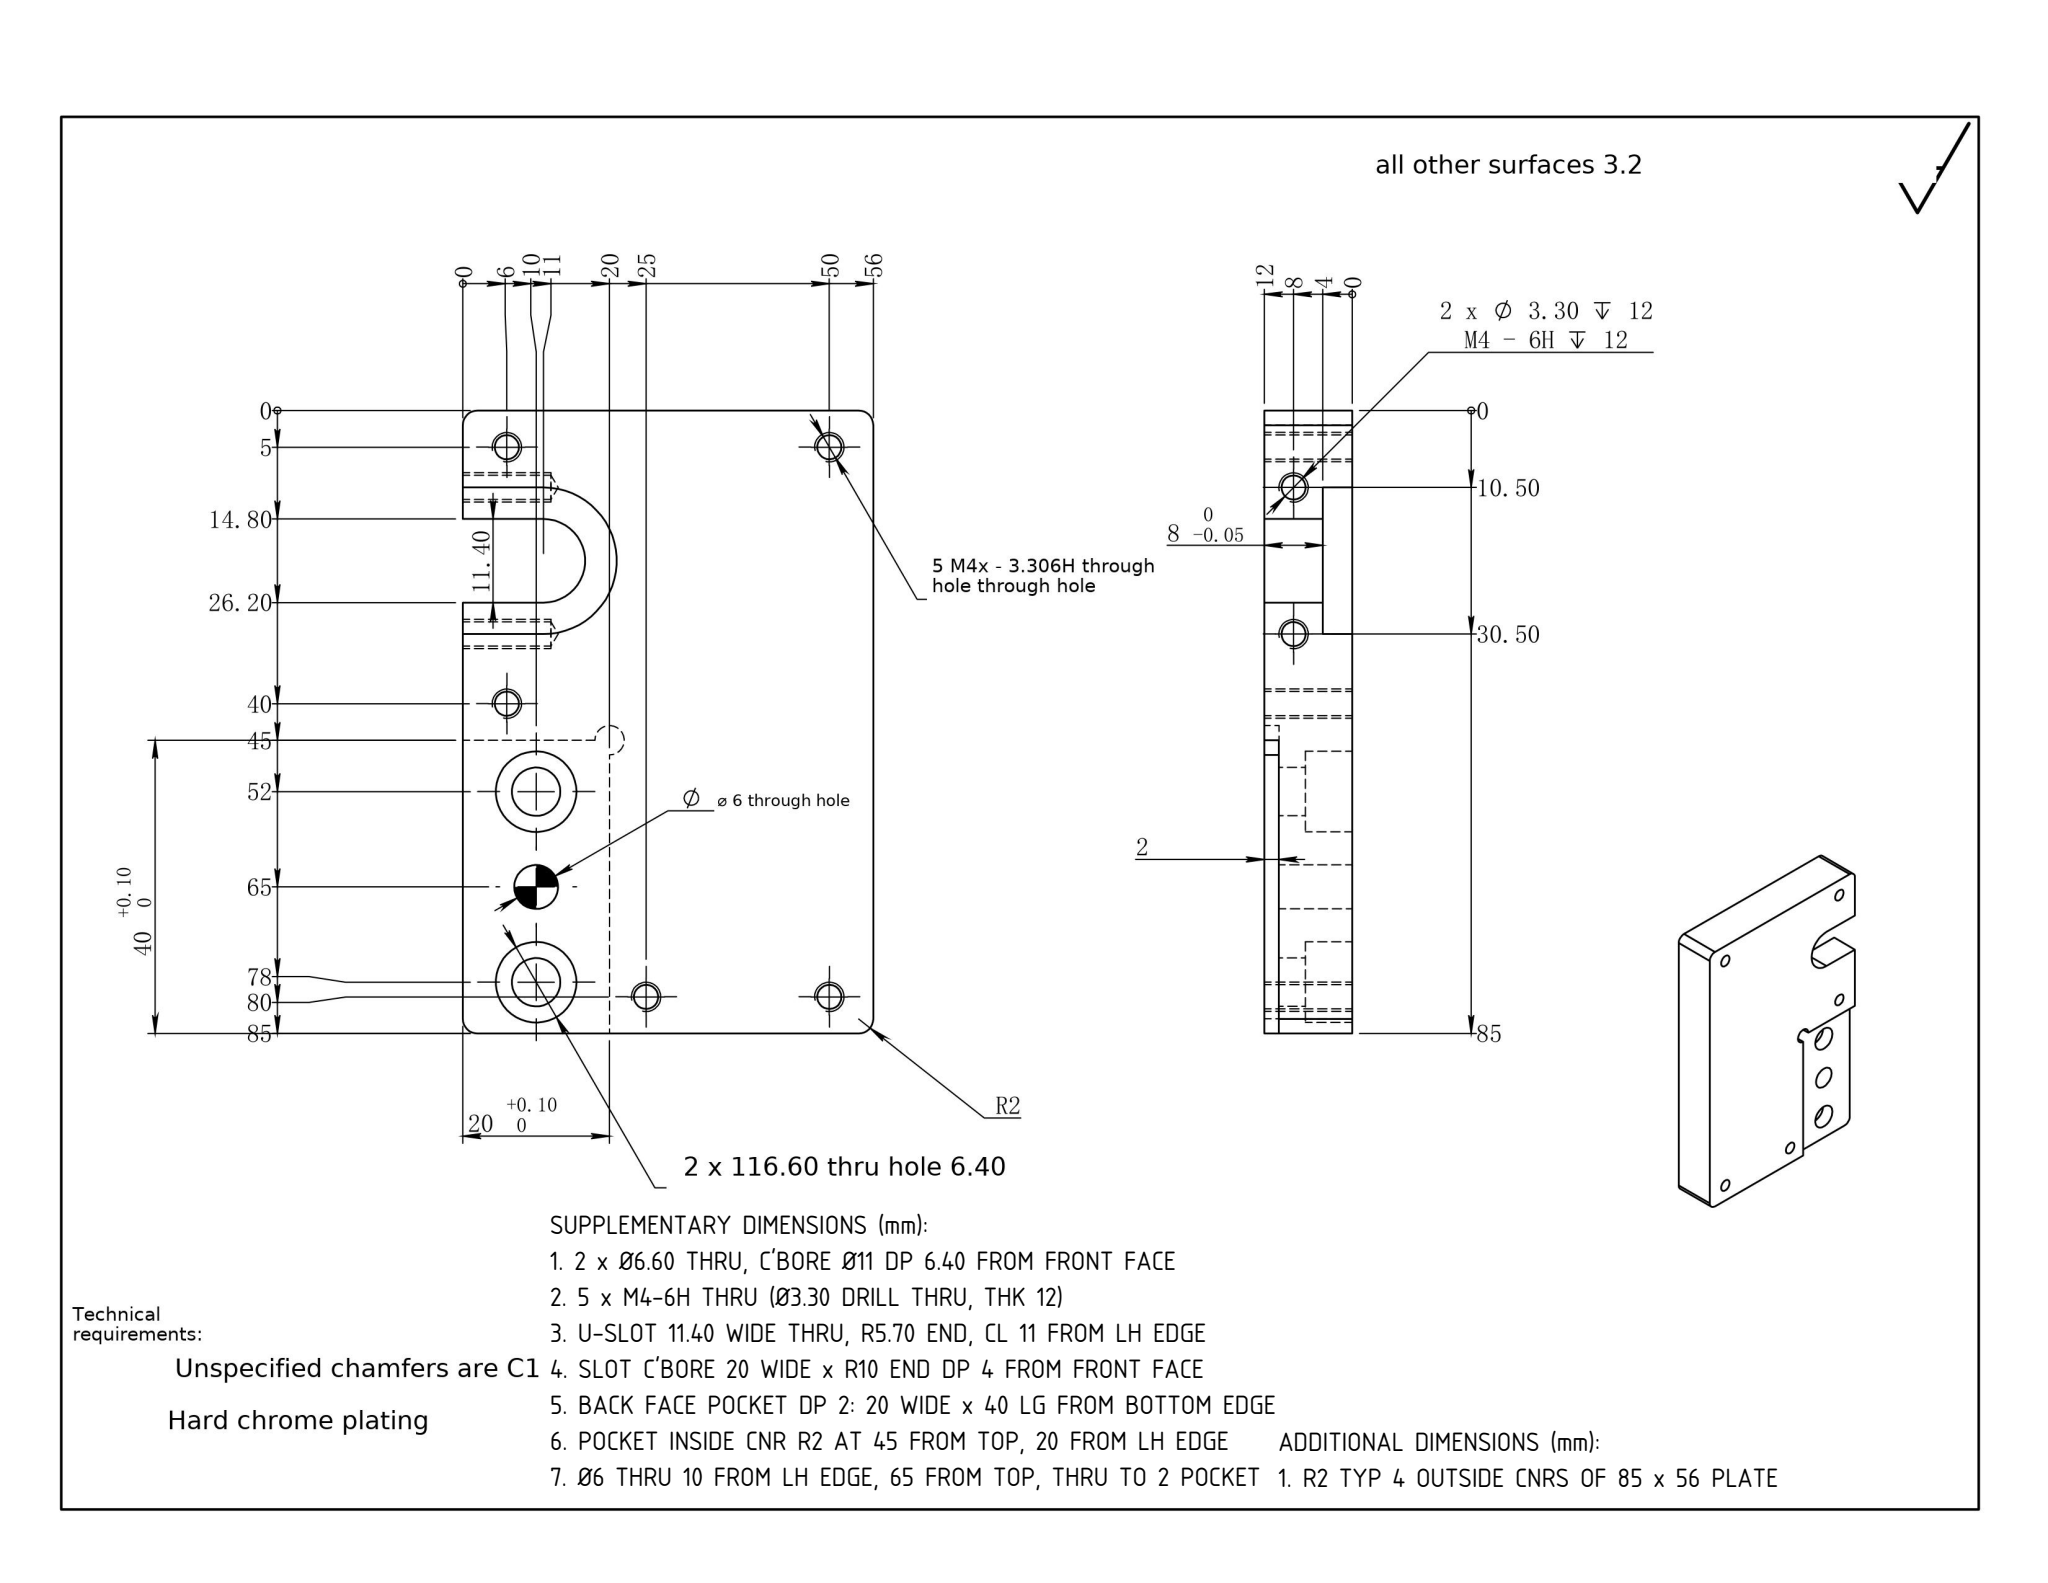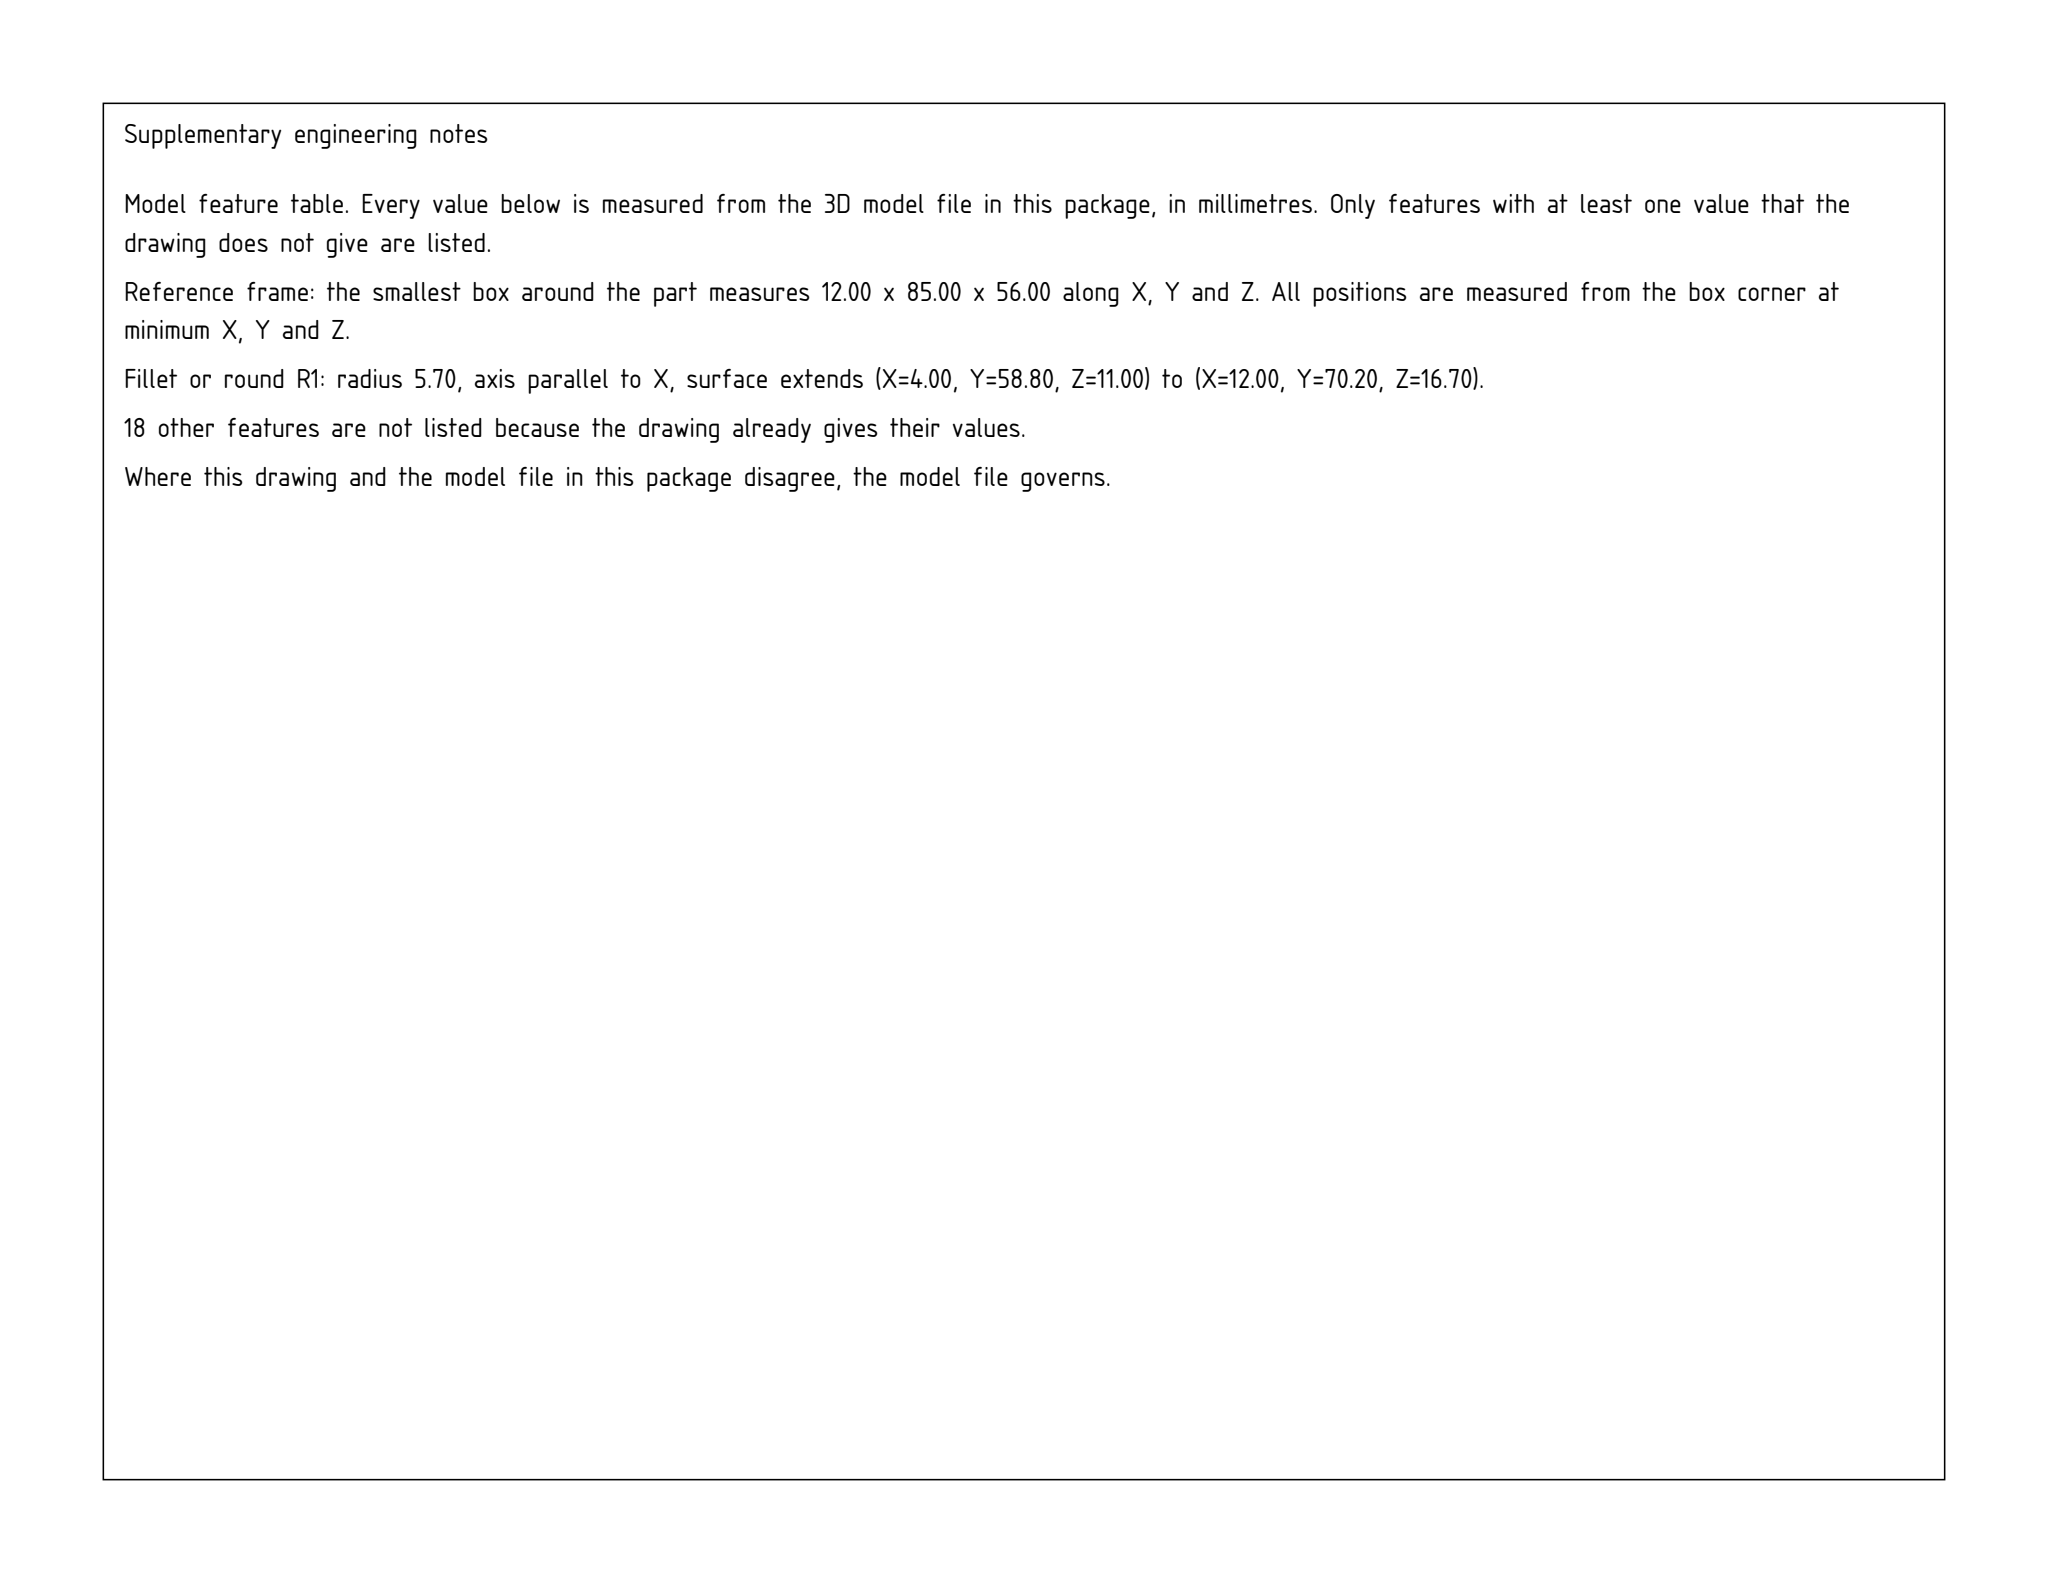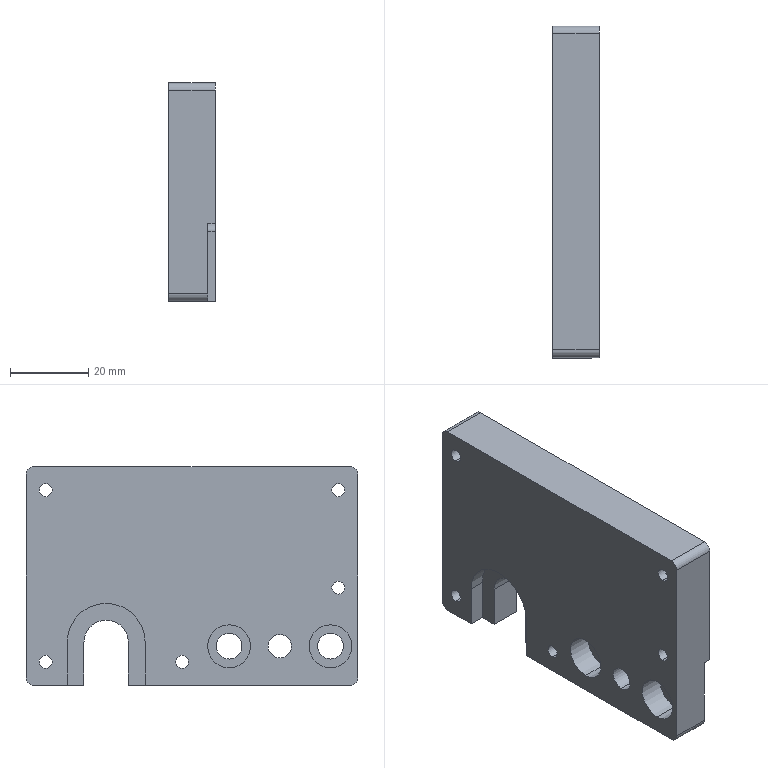Part | SolidWorks | mm | 1 solid | 55 faces | box 12 x 85 x 56 mm | volume 50072 mm3 | cylinder 34 | plane 17 | cone 4 | commonest cylinder face diameters 3.3 x14 4 x6 11 x4 6.6 x4 20 x2 6 x2 11.4 x2
build123d program:
from build123d import *

# Parameters (mm, degrees)
SKETCH1_W                                       = 56
SKETCH1_H                                       = 85
BOSS_EXTRUDE1_DEPTH                             = 12
M6_HEX_SOCKET_HEAD_CAP_SCREW_CBORE1_D           = 6.6
M6_HEX_SOCKET_HEAD_CAP_SCREW_CBORE1_CBORE_D     = 11
M6_HEX_SOCKET_HEAD_CAP_SCREW_CBORE1_CBORE_DEPTH = 6.4
F_6_0_6_DIAMETER_HOLE1_D                        = 6
SKETCH10_W                                      = 20
SKETCH10_H                                      = 40
CUT_EXTRUDE1_DEPTH                              = 2
SKETCH11_R                                      = 2
CUT_EXTRUDE2_DEPTH                              = 52.868
SKETCH12_R                                      = 5.7
CUT_EXTRUDE3_DEPTH                              = 53.29
CUT_EXTRUDE4_DEPTH                              = 4
CUT_EXTRUDE5_DEPTH                              = 52.519
M4_TAPPED_HOLE1_D                               = 3.3
FILLET1_R                                       = 2
M4_TAPPED_HOLE2_D                               = 3.3
M4_TAPPED_HOLE2_DEPTH                           = 12
M4_TAPPED_HOLE2_TIP                             = 0.9914


with BuildPart() as part:
    # Sketch1 → Boss-Extrude1 (new body)
    with BuildSketch(Plane(origin=(0, 0, 0), x_dir=(0, 0, -1), z_dir=(1, 0, 0))):
        Rectangle(SKETCH1_W, SKETCH1_H)
    extrude(amount=BOSS_EXTRUDE1_DEPTH)

    # M6 Hex Socket Head Cap Screw CBORE1 (through all)
    with Locations(Plane.ZY):
        with Locations((-18, -9.5), (-18, -35.5)):
            CounterBoreHole(M6_HEX_SOCKET_HEAD_CAP_SCREW_CBORE1_D / 2, M6_HEX_SOCKET_HEAD_CAP_SCREW_CBORE1_CBORE_D / 2, M6_HEX_SOCKET_HEAD_CAP_SCREW_CBORE1_CBORE_DEPTH)

    # 6.0 _6_ Diameter Hole1 (through all)
    with Locations(Plane(origin=(12, 0, 0), x_dir=(0, 0, -1), z_dir=(1, 0, 0))):
        with Locations((18, -22.5)):
            Hole(F_6_0_6_DIAMETER_HOLE1_D / 2)

    # Sketch10 → Cut-Extrude1 (cut)
    with BuildSketch(Plane(origin=(12, 0, 0), x_dir=(0, 0, -1), z_dir=(1, 0, 0))):
        with Locations((18, -22.5)):
            Rectangle(SKETCH10_W, SKETCH10_H)
    extrude(amount=-CUT_EXTRUDE1_DEPTH, mode=Mode.SUBTRACT)

    # Sketch11 → Cut-Extrude2 (cut, through all)
    with BuildSketch(Plane(origin=(10, 0, 0), x_dir=(0, 0, -1), z_dir=(1, 0, 0))):
        with Locations((8, -2.5)):
            Circle(SKETCH11_R)
    extrude(amount=CUT_EXTRUDE2_DEPTH, mode=Mode.SUBTRACT)

    # Sketch12 → Cut-Extrude3 (cut, through all)
    with BuildSketch(Plane.ZY):
        with Locations((-17, 22)):
            Circle(SKETCH12_R)
    extrude(amount=-CUT_EXTRUDE3_DEPTH, mode=Mode.SUBTRACT)

    # Sketch13 → Cut-Extrude4 (cut)
    with BuildSketch(Plane.ZY):
        with BuildLine():
            Line((-17, 12), (-28, 12))
            ThreePointArc((-28, 12), (-38, 22), (-28, 32))
            Line((-28, 32), (-17, 32))
            ThreePointArc((-17, 32), (-7, 22), (-17, 12))
        make_face()
    extrude(amount=-CUT_EXTRUDE4_DEPTH, mode=Mode.SUBTRACT)

    # Sketch14 → Cut-Extrude5 (cut, through all)
    with BuildSketch(Plane.ZY.offset(-4)):
        with BuildLine():
            Line((-28, 27.7), (-17, 27.7))
            ThreePointArc((-17, 27.7), (-11.3, 22), (-17, 16.3))
            Line((-17, 16.3), (-28, 16.3))
            ThreePointArc((-28, 16.3), (-33.7, 22), (-28, 27.7))
        make_face()
    extrude(amount=-CUT_EXTRUDE5_DEPTH, mode=Mode.SUBTRACT)

    # M4 Tapped Hole1 (through all)
    with Locations(Plane.ZY):
        with Locations((22, 37.5), (22, -37.5), (-22, 2.5), (-22, 37.5), (-3, -37.5)):
            Hole(M4_TAPPED_HOLE1_D / 2)

    # Fillet1
    fillet1_edges = [part.edges().sort_by_distance(p)[0] for p in [
        (5, -42.5, -28),
        (6, -42.5, 28),
        (6, 42.5, 28),
        (6, 42.5, -28),
    ]]
    fillet(fillet1_edges, radius=FILLET1_R)

    # M4 Tapped Hole2
    with Locations(Plane(origin=(0, 0, -28), x_dir=(-1, 0, 0), z_dir=(0, 0, -1))):
        with Locations((-8, 32), (-8, 12)):
            Hole(M4_TAPPED_HOLE2_D / 2, depth=M4_TAPPED_HOLE2_DEPTH)
            with Locations((0, 0, -(M4_TAPPED_HOLE2_DEPTH + M4_TAPPED_HOLE2_TIP / 2))):  # 118° drill point
                Cone(0, M4_TAPPED_HOLE2_D / 2, M4_TAPPED_HOLE2_TIP, mode=Mode.SUBTRACT)


solid = part.part